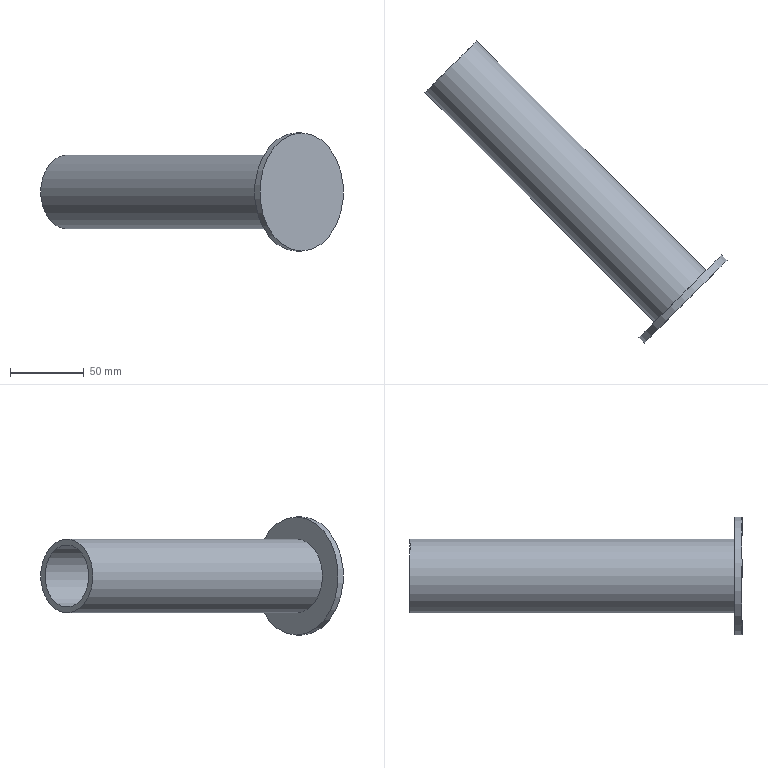Component | NX | SLID_FRAME_SUPP_COL | 1 solid | 7 faces | box 205.06 x 205.06 x 80 mm | volume 150919 mm3 | plane 4 | cylinder 3 | commonest cylinder face diameters 80 x1 50 x1 42 x1
STEP:
#1=CARTESIAN_POINT('',(0.,0.,0.));
#2=DIRECTION('',(0.,0.,1.));
#3=DIRECTION('',(1.,0.,0.));
#4=AXIS2_PLACEMENT_3D('',#1,#2,#3);
#5=CARTESIAN_POINT('',(-903.75,1528.914,235.));
#6=VERTEX_POINT('',#5);
#7=CARTESIAN_POINT('',(-903.75,1528.914,260.));
#8=DIRECTION('',(-0.7071,0.7071,0.));
#9=DIRECTION('',(0.,0.,-1.));
#10=AXIS2_PLACEMENT_3D('',#7,#8,#9);
#11=CIRCLE('',#10,25.);
#12=CARTESIAN_POINT('',(-903.75,1528.914,260.));
#13=DIRECTION('',(-0.7071,0.7071,0.));
#14=DIRECTION('',(0.,0.,-1.));
#15=AXIS2_PLACEMENT_3D('',#12,#13,#14);
#16=PLANE('',#15);
#17=CARTESIAN_POINT('',(0.,0.));
#18=DIRECTION('',(1.,0.));
#19=AXIS2_PLACEMENT_2D('',#17,#18);
#20=CIRCLE('',#19,25.);
#21=(GEOMETRIC_REPRESENTATION_CONTEXT(2)PARAMETRIC_REPRESENTATION_CONTEXT()REPRESENTATION_CONTEXT('',''));
#22=DEFINITIONAL_REPRESENTATION('',(#20),#21);
#23=PCURVE('',#16,#22);
#24=CARTESIAN_POINT('',(-903.75,1528.914,260.));
#25=DIRECTION('',(-0.7071,0.7071,0.));
#26=DIRECTION('',(0.,0.,-1.));
#27=AXIS2_PLACEMENT_3D('',#24,#25,#26);
#28=CYLINDRICAL_SURFACE('',#27,25.);
#29=CARTESIAN_POINT('',(0.,0.));
#30=DIRECTION('',(1.,0.));
#31=VECTOR('',#30,1.);
#32=LINE('',#29,#31);
#33=(GEOMETRIC_REPRESENTATION_CONTEXT(2)PARAMETRIC_REPRESENTATION_CONTEXT()REPRESENTATION_CONTEXT('',''));
#34=DEFINITIONAL_REPRESENTATION('',(#32),#33);
#35=PCURVE('',#28,#34);
#36=SURFACE_CURVE('',#11,(#23,#35),.PCURVE_S1.);
#37=EDGE_CURVE('',#6,#6,#36,.T.);
#38=ORIENTED_EDGE('',*,*,#37,.F.);
#39=EDGE_LOOP('',(#38));
#40=FACE_BOUND('',#39,.T.);
#41=CARTESIAN_POINT('',(-903.75,1528.914,220.));
#42=VERTEX_POINT('',#41);
#43=CARTESIAN_POINT('',(-903.75,1528.914,260.));
#44=DIRECTION('',(0.7071,-0.7071,0.));
#45=DIRECTION('',(0.,0.,-1.));
#46=AXIS2_PLACEMENT_3D('',#43,#44,#45);
#47=CIRCLE('',#46,40.);
#48=CARTESIAN_POINT('',(40.,0.));
#49=CARTESIAN_POINT('',(40.,-69.282));
#50=CARTESIAN_POINT('',(-20.,-34.641));
#51=CARTESIAN_POINT('',(-80.,-0.));
#52=CARTESIAN_POINT('',(-20.,34.641));
#53=CARTESIAN_POINT('',(40.,69.282));
#54=CARTESIAN_POINT('',(40.,0.));
#55=(BOUNDED_CURVE()B_SPLINE_CURVE(2,(#48,#49,#50,#51,#52,#53,#54),.UNSPECIFIED.,.T.,.F.)B_SPLINE_CURVE_WITH_KNOTS((1,2,2,2,2,1),(-2.094,0.,2.094,4.189,6.283,8.378),.UNSPECIFIED.)CURVE()GEOMETRIC_REPRESENTATION_ITEM()RATIONAL_B_SPLINE_CURVE((1.,0.5,1.,0.5,1.,0.5,1.))REPRESENTATION_ITEM(''));
#56=(GEOMETRIC_REPRESENTATION_CONTEXT(2)PARAMETRIC_REPRESENTATION_CONTEXT()REPRESENTATION_CONTEXT('',''));
#57=DEFINITIONAL_REPRESENTATION('',(#55),#56);
#58=PCURVE('',#16,#57);
#59=CARTESIAN_POINT('',(-900.214,1525.378,260.));
#60=DIRECTION('',(-0.7071,0.7071,0.));
#61=DIRECTION('',(0.,0.,-1.));
#62=AXIS2_PLACEMENT_3D('',#59,#60,#61);
#63=CYLINDRICAL_SURFACE('',#62,40.);
#64=CARTESIAN_POINT('',(6.283,5.));
#65=DIRECTION('',(-1.,0.));
#66=VECTOR('',#65,1.);
#67=LINE('',#64,#66);
#68=(GEOMETRIC_REPRESENTATION_CONTEXT(2)PARAMETRIC_REPRESENTATION_CONTEXT()REPRESENTATION_CONTEXT('',''));
#69=DEFINITIONAL_REPRESENTATION('',(#67),#68);
#70=PCURVE('',#63,#69);
#71=SURFACE_CURVE('',#47,(#58,#70),.PCURVE_S1.);
#72=EDGE_CURVE('',#42,#42,#71,.T.);
#73=ORIENTED_EDGE('',*,*,#72,.F.);
#74=EDGE_LOOP('',(#73));
#75=FACE_BOUND('',#74,.T.);
#76=ADVANCED_FACE('',(#40,#75),#16,.T.);
#77=CARTESIAN_POINT('',(-900.214,1525.378,220.));
#78=VERTEX_POINT('',#77);
#79=CARTESIAN_POINT('',(-900.214,1525.378,260.));
#80=DIRECTION('',(-0.7071,0.7071,0.));
#81=DIRECTION('',(0.,0.,-1.));
#82=AXIS2_PLACEMENT_3D('',#79,#80,#81);
#83=CIRCLE('',#82,40.);
#84=CARTESIAN_POINT('',(-900.214,1525.378,260.));
#85=DIRECTION('',(0.7071,-0.7071,0.));
#86=DIRECTION('',(0.,0.,1.));
#87=AXIS2_PLACEMENT_3D('',#84,#85,#86);
#88=PLANE('',#87);
#89=CARTESIAN_POINT('',(-40.,0.));
#90=CARTESIAN_POINT('',(-40.,69.282));
#91=CARTESIAN_POINT('',(20.,34.641));
#92=CARTESIAN_POINT('',(80.,0.));
#93=CARTESIAN_POINT('',(20.,-34.641));
#94=CARTESIAN_POINT('',(-40.,-69.282));
#95=CARTESIAN_POINT('',(-40.,0.));
#96=(BOUNDED_CURVE()B_SPLINE_CURVE(2,(#89,#90,#91,#92,#93,#94,#95),.UNSPECIFIED.,.T.,.F.)B_SPLINE_CURVE_WITH_KNOTS((1,2,2,2,2,1),(-2.094,0.,2.094,4.189,6.283,8.378),.UNSPECIFIED.)CURVE()GEOMETRIC_REPRESENTATION_ITEM()RATIONAL_B_SPLINE_CURVE((1.,0.5,1.,0.5,1.,0.5,1.))REPRESENTATION_ITEM(''));
#97=(GEOMETRIC_REPRESENTATION_CONTEXT(2)PARAMETRIC_REPRESENTATION_CONTEXT()REPRESENTATION_CONTEXT('',''));
#98=DEFINITIONAL_REPRESENTATION('',(#96),#97);
#99=PCURVE('',#88,#98);
#100=CARTESIAN_POINT('',(0.,0.));
#101=DIRECTION('',(1.,0.));
#102=VECTOR('',#101,1.);
#103=LINE('',#100,#102);
#104=(GEOMETRIC_REPRESENTATION_CONTEXT(2)PARAMETRIC_REPRESENTATION_CONTEXT()REPRESENTATION_CONTEXT('',''));
#105=DEFINITIONAL_REPRESENTATION('',(#103),#104);
#106=PCURVE('',#63,#105);
#107=SURFACE_CURVE('',#83,(#99,#106),.PCURVE_S1.);
#108=EDGE_CURVE('',#78,#78,#107,.T.);
#109=ORIENTED_EDGE('',*,*,#108,.F.);
#110=EDGE_LOOP('',(#109));
#111=FACE_BOUND('',#110,.T.);
#112=ADVANCED_FACE('',(#111),#88,.T.);
#113=ORIENTED_EDGE('',*,*,#72,.T.);
#114=CARTESIAN_POINT('',(-900.214,1525.378,220.));
#115=CARTESIAN_POINT('',(-903.75,1528.914,220.));
#116=B_SPLINE_CURVE_WITH_KNOTS('',1,(#114,#115),.UNSPECIFIED.,.F.,.F.,(2,2),(0.,5.),.PIECEWISE_BEZIER_KNOTS.);
#117=CARTESIAN_POINT('',(0.,0.));
#118=DIRECTION('',(0.,1.));
#119=VECTOR('',#118,1.);
#120=LINE('',#117,#119);
#121=(GEOMETRIC_REPRESENTATION_CONTEXT(2)PARAMETRIC_REPRESENTATION_CONTEXT()REPRESENTATION_CONTEXT('',''));
#122=DEFINITIONAL_REPRESENTATION('',(#120),#121);
#123=PCURVE('',#63,#122);
#124=CARTESIAN_POINT('',(6.283,0.));
#125=DIRECTION('',(0.,1.));
#126=VECTOR('',#125,1.);
#127=LINE('',#124,#126);
#128=(GEOMETRIC_REPRESENTATION_CONTEXT(2)PARAMETRIC_REPRESENTATION_CONTEXT()REPRESENTATION_CONTEXT('',''));
#129=DEFINITIONAL_REPRESENTATION('',(#127),#128);
#130=PCURVE('',#63,#129);
#131=SEAM_CURVE('',#116,(#123,#130),.PCURVE_S1.);
#132=EDGE_CURVE('',#78,#42,#131,.T.);
#133=ORIENTED_EDGE('',*,*,#132,.F.);
#134=ORIENTED_EDGE('',*,*,#108,.T.);
#135=ORIENTED_EDGE('',*,*,#132,.T.);
#136=EDGE_LOOP('',(#113,#133,#134,#135));
#137=FACE_BOUND('',#136,.T.);
#138=ADVANCED_FACE('',(#137),#63,.T.);
#139=CARTESIAN_POINT('',(-1059.313,1684.477,239.));
#140=VERTEX_POINT('',#139);
#141=CARTESIAN_POINT('',(-1059.313,1684.477,260.));
#142=DIRECTION('',(-0.7071,0.7071,0.));
#143=DIRECTION('',(0.,0.,-1.));
#144=AXIS2_PLACEMENT_3D('',#141,#142,#143);
#145=CIRCLE('',#144,21.);
#146=CARTESIAN_POINT('',(-1059.313,1684.477,260.));
#147=DIRECTION('',(-0.7071,0.7071,0.));
#148=DIRECTION('',(0.,0.,-1.));
#149=AXIS2_PLACEMENT_3D('',#146,#147,#148);
#150=PLANE('',#149);
#151=CARTESIAN_POINT('',(0.,0.));
#152=DIRECTION('',(1.,0.));
#153=AXIS2_PLACEMENT_2D('',#151,#152);
#154=CIRCLE('',#153,21.);
#155=(GEOMETRIC_REPRESENTATION_CONTEXT(2)PARAMETRIC_REPRESENTATION_CONTEXT()REPRESENTATION_CONTEXT('',''));
#156=DEFINITIONAL_REPRESENTATION('',(#154),#155);
#157=PCURVE('',#150,#156);
#158=CARTESIAN_POINT('',(-903.75,1528.914,260.));
#159=DIRECTION('',(-0.7071,0.7071,0.));
#160=DIRECTION('',(0.,0.,-1.));
#161=AXIS2_PLACEMENT_3D('',#158,#159,#160);
#162=CYLINDRICAL_SURFACE('',#161,21.);
#163=CARTESIAN_POINT('',(0.,220.));
#164=DIRECTION('',(1.,0.));
#165=VECTOR('',#164,1.);
#166=LINE('',#163,#165);
#167=(GEOMETRIC_REPRESENTATION_CONTEXT(2)PARAMETRIC_REPRESENTATION_CONTEXT()REPRESENTATION_CONTEXT('',''));
#168=DEFINITIONAL_REPRESENTATION('',(#166),#167);
#169=PCURVE('',#162,#168);
#170=SURFACE_CURVE('',#145,(#157,#169),.PCURVE_S1.);
#171=EDGE_CURVE('',#140,#140,#170,.T.);
#172=ORIENTED_EDGE('',*,*,#171,.F.);
#173=EDGE_LOOP('',(#172));
#174=FACE_BOUND('',#173,.T.);
#175=CARTESIAN_POINT('',(-1059.313,1684.477,235.));
#176=VERTEX_POINT('',#175);
#177=CARTESIAN_POINT('',(-1059.313,1684.477,260.));
#178=DIRECTION('',(-0.7071,0.7071,0.));
#179=DIRECTION('',(0.,0.,-1.));
#180=AXIS2_PLACEMENT_3D('',#177,#178,#179);
#181=CIRCLE('',#180,25.);
#182=CARTESIAN_POINT('',(0.,0.));
#183=DIRECTION('',(1.,0.));
#184=AXIS2_PLACEMENT_2D('',#182,#183);
#185=CIRCLE('',#184,25.);
#186=(GEOMETRIC_REPRESENTATION_CONTEXT(2)PARAMETRIC_REPRESENTATION_CONTEXT()REPRESENTATION_CONTEXT('',''));
#187=DEFINITIONAL_REPRESENTATION('',(#185),#186);
#188=PCURVE('',#150,#187);
#189=CARTESIAN_POINT('',(0.,220.));
#190=DIRECTION('',(1.,0.));
#191=VECTOR('',#190,1.);
#192=LINE('',#189,#191);
#193=(GEOMETRIC_REPRESENTATION_CONTEXT(2)PARAMETRIC_REPRESENTATION_CONTEXT()REPRESENTATION_CONTEXT('',''));
#194=DEFINITIONAL_REPRESENTATION('',(#192),#193);
#195=PCURVE('',#28,#194);
#196=SURFACE_CURVE('',#181,(#188,#195),.PCURVE_S1.);
#197=EDGE_CURVE('',#176,#176,#196,.T.);
#198=ORIENTED_EDGE('',*,*,#197,.T.);
#199=EDGE_LOOP('',(#198));
#200=FACE_BOUND('',#199,.T.);
#201=ADVANCED_FACE('',(#174,#200),#150,.T.);
#202=ORIENTED_EDGE('',*,*,#197,.F.);
#203=CARTESIAN_POINT('',(-903.75,1528.914,235.));
#204=CARTESIAN_POINT('',(-1059.313,1684.477,235.));
#205=B_SPLINE_CURVE_WITH_KNOTS('',1,(#203,#204),.UNSPECIFIED.,.F.,.F.,(2,2),(0.,220.),.PIECEWISE_BEZIER_KNOTS.);
#206=CARTESIAN_POINT('',(0.,0.));
#207=DIRECTION('',(0.,1.));
#208=VECTOR('',#207,1.);
#209=LINE('',#206,#208);
#210=(GEOMETRIC_REPRESENTATION_CONTEXT(2)PARAMETRIC_REPRESENTATION_CONTEXT()REPRESENTATION_CONTEXT('',''));
#211=DEFINITIONAL_REPRESENTATION('',(#209),#210);
#212=PCURVE('',#28,#211);
#213=CARTESIAN_POINT('',(6.283,0.));
#214=DIRECTION('',(0.,1.));
#215=VECTOR('',#214,1.);
#216=LINE('',#213,#215);
#217=(GEOMETRIC_REPRESENTATION_CONTEXT(2)PARAMETRIC_REPRESENTATION_CONTEXT()REPRESENTATION_CONTEXT('',''));
#218=DEFINITIONAL_REPRESENTATION('',(#216),#217);
#219=PCURVE('',#28,#218);
#220=SEAM_CURVE('',#205,(#212,#219),.PCURVE_S1.);
#221=EDGE_CURVE('',#6,#176,#220,.T.);
#222=ORIENTED_EDGE('',*,*,#221,.F.);
#223=ORIENTED_EDGE('',*,*,#37,.T.);
#224=ORIENTED_EDGE('',*,*,#221,.T.);
#225=EDGE_LOOP('',(#202,#222,#223,#224));
#226=FACE_BOUND('',#225,.T.);
#227=ADVANCED_FACE('',(#226),#28,.T.);
#228=CARTESIAN_POINT('',(-903.043,1528.207,281.));
#229=VERTEX_POINT('',#228);
#230=CARTESIAN_POINT('',(-903.043,1528.207,239.));
#231=VERTEX_POINT('',#230);
#232=CARTESIAN_POINT('',(-903.043,1528.207,260.));
#233=DIRECTION('',(0.7071,-0.7071,0.));
#234=DIRECTION('',(0.,0.,1.));
#235=AXIS2_PLACEMENT_3D('',#232,#233,#234);
#236=CIRCLE('',#235,21.);
#237=CARTESIAN_POINT('',(-903.043,1528.207,260.));
#238=DIRECTION('',(0.7071,-0.7071,0.));
#239=DIRECTION('',(0.,0.,1.));
#240=AXIS2_PLACEMENT_3D('',#237,#238,#239);
#241=PLANE('',#240);
#242=CARTESIAN_POINT('',(0.,0.));
#243=DIRECTION('',(1.,0.));
#244=AXIS2_PLACEMENT_2D('',#242,#243);
#245=CIRCLE('',#244,21.);
#246=(GEOMETRIC_REPRESENTATION_CONTEXT(2)PARAMETRIC_REPRESENTATION_CONTEXT()REPRESENTATION_CONTEXT('',''));
#247=DEFINITIONAL_REPRESENTATION('',(#245),#246);
#248=PCURVE('',#241,#247);
#249=CARTESIAN_POINT('',(3.142,-1.));
#250=DIRECTION('',(-1.,0.));
#251=VECTOR('',#250,1.);
#252=LINE('',#249,#251);
#253=(GEOMETRIC_REPRESENTATION_CONTEXT(2)PARAMETRIC_REPRESENTATION_CONTEXT()REPRESENTATION_CONTEXT('',''));
#254=DEFINITIONAL_REPRESENTATION('',(#252),#253);
#255=PCURVE('',#162,#254);
#256=SURFACE_CURVE('',#236,(#248,#255),.PCURVE_S1.);
#257=EDGE_CURVE('',#229,#231,#256,.T.);
#258=ORIENTED_EDGE('',*,*,#257,.F.);
#259=CARTESIAN_POINT('',(-903.043,1528.207,260.));
#260=DIRECTION('',(0.7071,-0.7071,0.));
#261=DIRECTION('',(0.,0.,1.));
#262=AXIS2_PLACEMENT_3D('',#259,#260,#261);
#263=CIRCLE('',#262,21.);
#264=CARTESIAN_POINT('',(0.,0.));
#265=DIRECTION('',(1.,0.));
#266=AXIS2_PLACEMENT_2D('',#264,#265);
#267=CIRCLE('',#266,21.);
#268=(GEOMETRIC_REPRESENTATION_CONTEXT(2)PARAMETRIC_REPRESENTATION_CONTEXT()REPRESENTATION_CONTEXT('',''));
#269=DEFINITIONAL_REPRESENTATION('',(#267),#268);
#270=PCURVE('',#241,#269);
#271=CARTESIAN_POINT('',(9.425,-1.));
#272=DIRECTION('',(-1.,0.));
#273=VECTOR('',#272,1.);
#274=LINE('',#271,#273);
#275=(GEOMETRIC_REPRESENTATION_CONTEXT(2)PARAMETRIC_REPRESENTATION_CONTEXT()REPRESENTATION_CONTEXT('',''));
#276=DEFINITIONAL_REPRESENTATION('',(#274),#275);
#277=PCURVE('',#162,#276);
#278=SURFACE_CURVE('',#263,(#270,#277),.PCURVE_S1.);
#279=EDGE_CURVE('',#231,#229,#278,.T.);
#280=ORIENTED_EDGE('',*,*,#279,.F.);
#281=EDGE_LOOP('',(#258,#280));
#282=FACE_BOUND('',#281,.T.);
#283=ADVANCED_FACE('',(#282),#241,.F.);
#284=ORIENTED_EDGE('',*,*,#279,.F.);
#285=CARTESIAN_POINT('',(-903.043,1528.207,239.));
#286=CARTESIAN_POINT('',(-1059.313,1684.477,239.));
#287=B_SPLINE_CURVE_WITH_KNOTS('',1,(#285,#286),.UNSPECIFIED.,.F.,.F.,(2,2),(-1.,220.),.PIECEWISE_BEZIER_KNOTS.);
#288=CARTESIAN_POINT('',(6.283,0.));
#289=DIRECTION('',(0.,1.));
#290=VECTOR('',#289,1.);
#291=LINE('',#288,#290);
#292=(GEOMETRIC_REPRESENTATION_CONTEXT(2)PARAMETRIC_REPRESENTATION_CONTEXT()REPRESENTATION_CONTEXT('',''));
#293=DEFINITIONAL_REPRESENTATION('',(#291),#292);
#294=PCURVE('',#162,#293);
#295=CARTESIAN_POINT('',(0.,0.));
#296=DIRECTION('',(0.,1.));
#297=VECTOR('',#296,1.);
#298=LINE('',#295,#297);
#299=(GEOMETRIC_REPRESENTATION_CONTEXT(2)PARAMETRIC_REPRESENTATION_CONTEXT()REPRESENTATION_CONTEXT('',''));
#300=DEFINITIONAL_REPRESENTATION('',(#298),#299);
#301=PCURVE('',#162,#300);
#302=SEAM_CURVE('',#287,(#294,#301),.PCURVE_S1.);
#303=EDGE_CURVE('',#231,#140,#302,.T.);
#304=ORIENTED_EDGE('',*,*,#303,.T.);
#305=ORIENTED_EDGE('',*,*,#171,.F.);
#306=ORIENTED_EDGE('',*,*,#303,.F.);
#307=ORIENTED_EDGE('',*,*,#257,.F.);
#308=EDGE_LOOP('',(#284,#304,#305,#306,#307));
#309=FACE_BOUND('',#308,.F.);
#310=ADVANCED_FACE('',(#309),#162,.F.);
#311=CLOSED_SHELL('',(#76,#112,#138,#201,#227,#283,#310));
#312=MANIFOLD_SOLID_BREP('',#311);
#313=(LENGTH_UNIT()NAMED_UNIT(*)SI_UNIT(.MILLI.,.METRE.));
#314=UNCERTAINTY_MEASURE_WITH_UNIT(LENGTH_MEASURE(0.000005),#313,'','');
#315=(NAMED_UNIT(*)PLANE_ANGLE_UNIT()SI_UNIT($,.RADIAN.));
#316=(NAMED_UNIT(*)SI_UNIT($,.STERADIAN.)SOLID_ANGLE_UNIT());
#317=(GEOMETRIC_REPRESENTATION_CONTEXT(3)GLOBAL_UNCERTAINTY_ASSIGNED_CONTEXT((#314))GLOBAL_UNIT_ASSIGNED_CONTEXT((#313,#315,#316))REPRESENTATION_CONTEXT('',''));
#318=ADVANCED_BREP_SHAPE_REPRESENTATION('',(#4,#312),#317);